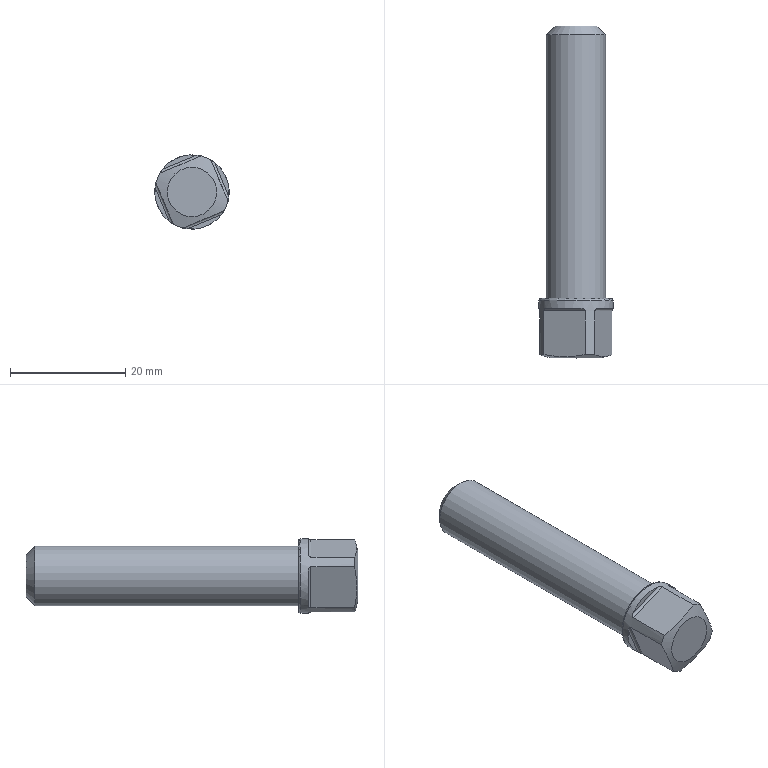Component | NX | SCREW | 1 solid | 20 faces | volume 5027 mm3 | plane 11 | cylinder 6 | cone 2 | torus 1 | commonest cylinder face diameters 0.86 x4 12.9 x1 10.32 x1